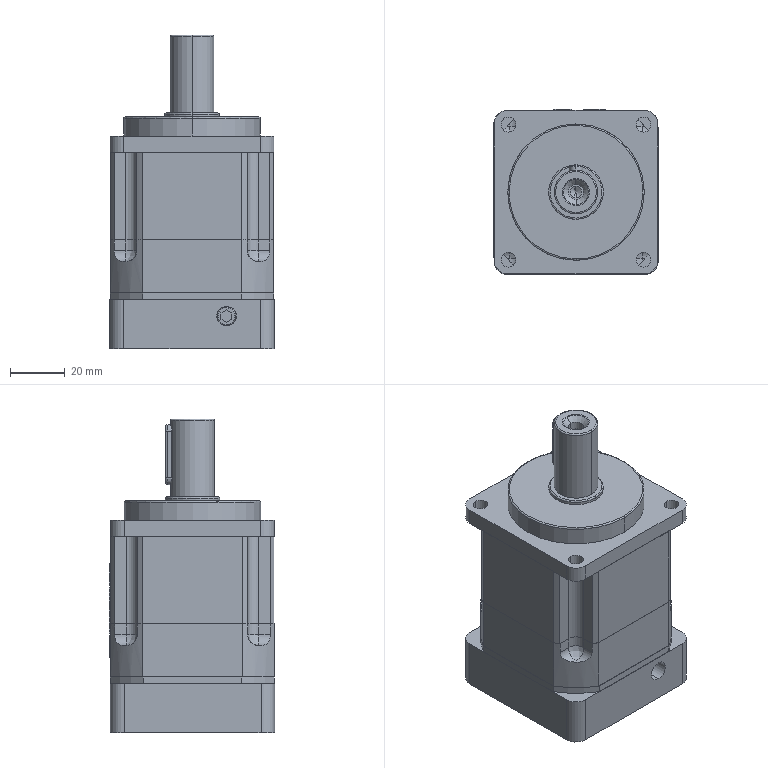Component | SolidWorks | Q1-A12-S21-Q1A.SLDASQ-1_Q1-PAB060-10-S2-P2-14-50-70-Q4-1 | 22 solids | 635 faces | volume 259399 mm3 | plane 427 | cylinder 98 | spline 96 | cone 14 | commonest cylinder face diameters 70 x16 8 x16 5.5 x14 10 x8 3.3 x8 7.2 x5 5 x5 40 x4